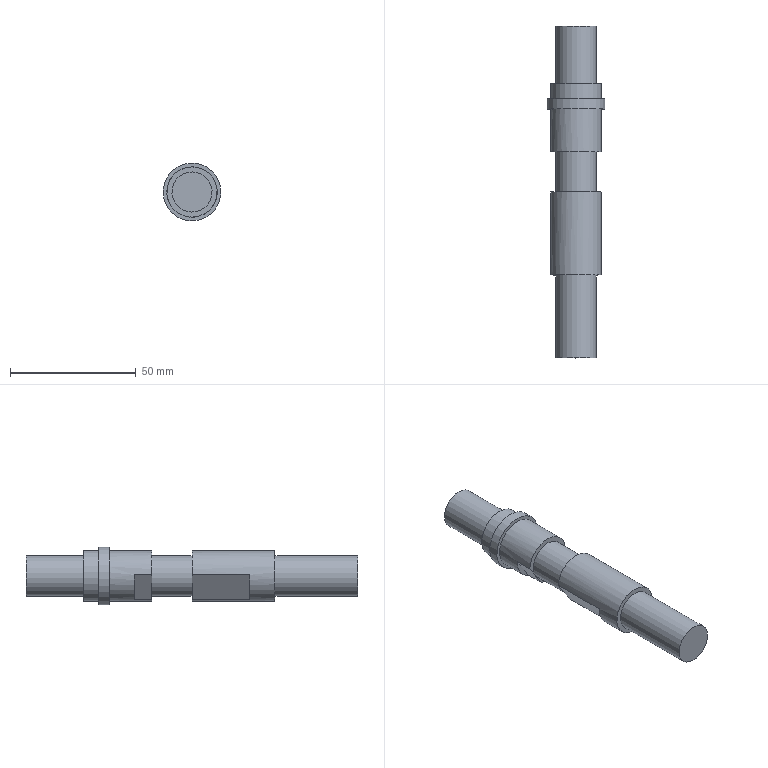Component | NX | MODEL7 | 1 solid | 19 faces | volume 33276 mm3 | plane 12 | cylinder 7 | commonest cylinder face diameters 20 x3 16 x3 23 x1